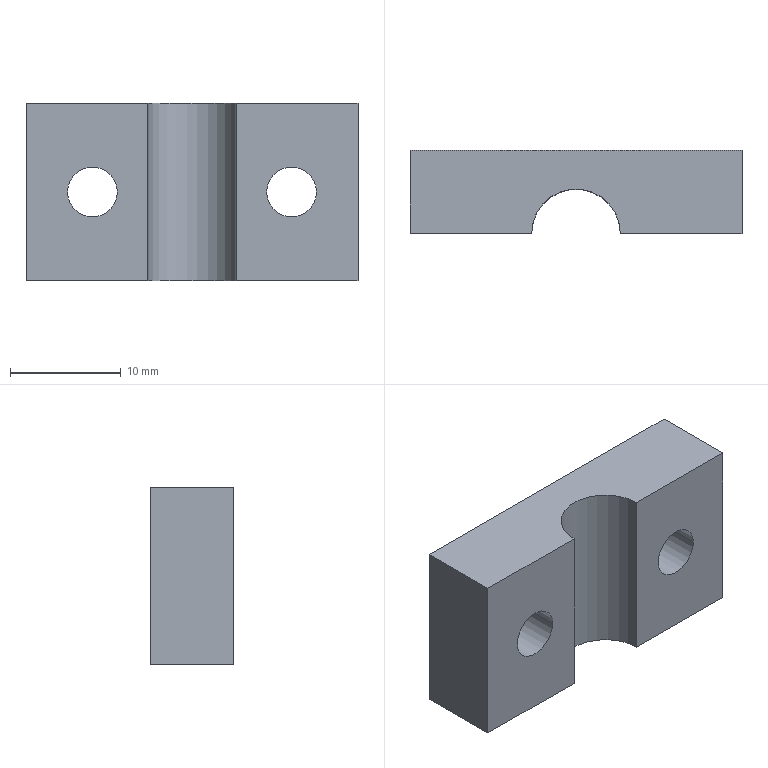Component | SolidWorks | JL001-05-03-1_JL001-05-01-012-1 | 1 solid | 12 faces | box 30 x 7.5 x 16 mm | volume 2959 mm3 | plane 7 | cylinder 5 | commonest cylinder face diameters 4.5 x4 8 x1
build123d program:
from build123d import *

# Parameters (mm, degrees)
SKETCH1_W                      = 16
SKETCH1_H                      = 30
BOSS_EXTRUDE1_DEPTH            = 7.5
SKETCH2_R                      = 4
CUT_EXTRUDE1_DEPTH             = 24.179
F_4_5_4_5_DIAMETER_HOLE1_D     = 4.5
F_4_5_4_5_DIAMETER_HOLE1_DEPTH = 10.1
F_4_5_4_5_DIAMETER_HOLE1_TIP   = 1.352


with BuildPart() as part:
    # Sketch1 → Boss-Extrude1 (new body)
    with BuildSketch(Plane(origin=(0, 0, 0), x_dir=(1, 0, 0), z_dir=(0, 1, 0))):
        Rectangle(SKETCH1_W, SKETCH1_H)
    extrude(amount=BOSS_EXTRUDE1_DEPTH)

    # Sketch2 → Cut-Extrude1 (cut, through all)
    with BuildSketch(Plane(origin=(8, 0, 0), x_dir=(0, 0, -1), z_dir=(1, 0, 0))):
        Circle(SKETCH2_R)
    extrude(amount=-CUT_EXTRUDE1_DEPTH, mode=Mode.SUBTRACT)

    # 4.5 _4.5_ Diameter Hole1
    with Locations(Plane(origin=(0, 7.5, 0), x_dir=(1, 0, 0), z_dir=(0, 1, 0))):
        with Locations((0, -9), (0, 9)):
            Hole(F_4_5_4_5_DIAMETER_HOLE1_D / 2, depth=F_4_5_4_5_DIAMETER_HOLE1_DEPTH)
            with Locations((0, 0, -(F_4_5_4_5_DIAMETER_HOLE1_DEPTH + F_4_5_4_5_DIAMETER_HOLE1_TIP / 2))):  # 118° drill point
                Cone(0, F_4_5_4_5_DIAMETER_HOLE1_D / 2, F_4_5_4_5_DIAMETER_HOLE1_TIP, mode=Mode.SUBTRACT)


solid = part.part

# Placed as in the assembly
solid = solid.moved(Location((0, 294.848, 85), (0, 90, 0)))
STEP:
#1=COLOUR_RGB('',0.7922,0.8196,0.9333);
#2=FILL_AREA_STYLE_COLOUR('',#1);
#3=FILL_AREA_STYLE('',(#2));
#4=SURFACE_STYLE_FILL_AREA(#3);
#5=SURFACE_SIDE_STYLE('',(#4));
#6=SURFACE_STYLE_USAGE(.BOTH.,#5);
#7=PRESENTATION_STYLE_ASSIGNMENT((#6));
#8=CARTESIAN_POINT('',(0.2657,11.608,3.346));
#9=VERTEX_POINT('',#8);
#10=CARTESIAN_POINT('',(0.4429,11.608,3.346));
#11=VERTEX_POINT('',#10);
#12=CARTESIAN_POINT('',(0.3543,11.608,3.346));
#13=DIRECTION('',(0.,1.,0.));
#14=DIRECTION('',(1.,0.,0.));
#15=AXIS2_PLACEMENT_3D('',#12,#13,#14);
#16=CIRCLE('',#15,0.08858);
#17=EDGE_CURVE('',#9,#11,#16,.T.);
#18=ORIENTED_EDGE('',*,*,#17,.F.);
#19=CARTESIAN_POINT('',(0.2657,11.903,3.346));
#20=VERTEX_POINT('',#19);
#21=CARTESIAN_POINT('',(0.2657,11.903,3.346));
#22=DIRECTION('',(0.,1.,0.));
#23=VECTOR('',#22,39.37);
#24=LINE('',#21,#23);
#25=EDGE_CURVE('',#9,#20,#24,.T.);
#26=ORIENTED_EDGE('',*,*,#25,.T.);
#27=CARTESIAN_POINT('',(0.4429,11.903,3.346));
#28=VERTEX_POINT('',#27);
#29=CARTESIAN_POINT('',(0.3543,11.903,3.346));
#30=DIRECTION('',(0.,1.,0.));
#31=DIRECTION('',(1.,0.,0.));
#32=AXIS2_PLACEMENT_3D('',#29,#30,#31);
#33=CIRCLE('',#32,0.08858);
#34=EDGE_CURVE('',#20,#28,#33,.T.);
#35=ORIENTED_EDGE('',*,*,#34,.T.);
#36=CARTESIAN_POINT('',(0.4429,11.903,3.346));
#37=DIRECTION('',(0.,1.,0.));
#38=VECTOR('',#37,39.37);
#39=LINE('',#36,#38);
#40=EDGE_CURVE('',#11,#28,#39,.T.);
#41=ORIENTED_EDGE('',*,*,#40,.F.);
#42=EDGE_LOOP('',(#18,#26,#35,#41));
#43=FACE_OUTER_BOUND('',#42,.T.);
#44=CARTESIAN_POINT('',(0.3543,11.903,3.346));
#45=DIRECTION('',(0.,1.,0.));
#46=DIRECTION('',(1.,0.,0.));
#47=AXIS2_PLACEMENT_3D('',#44,#45,#46);
#48=CYLINDRICAL_SURFACE('',#47,0.08858);
#49=ADVANCED_FACE('',(#43),#48,.F.);
#50=CARTESIAN_POINT('',(-0.4429,11.608,3.346));
#51=VERTEX_POINT('',#50);
#52=CARTESIAN_POINT('',(-0.2657,11.608,3.346));
#53=VERTEX_POINT('',#52);
#54=CARTESIAN_POINT('',(-0.3543,11.608,3.346));
#55=DIRECTION('',(0.,1.,0.));
#56=DIRECTION('',(1.,0.,0.));
#57=AXIS2_PLACEMENT_3D('',#54,#55,#56);
#58=CIRCLE('',#57,0.08858);
#59=EDGE_CURVE('',#51,#53,#58,.T.);
#60=ORIENTED_EDGE('',*,*,#59,.F.);
#61=CARTESIAN_POINT('',(-0.4429,11.903,3.346));
#62=VERTEX_POINT('',#61);
#63=CARTESIAN_POINT('',(-0.4429,11.903,3.346));
#64=DIRECTION('',(0.,1.,0.));
#65=VECTOR('',#64,39.37);
#66=LINE('',#63,#65);
#67=EDGE_CURVE('',#51,#62,#66,.T.);
#68=ORIENTED_EDGE('',*,*,#67,.T.);
#69=CARTESIAN_POINT('',(-0.2657,11.903,3.346));
#70=VERTEX_POINT('',#69);
#71=CARTESIAN_POINT('',(-0.3543,11.903,3.346));
#72=DIRECTION('',(0.,1.,0.));
#73=DIRECTION('',(1.,0.,0.));
#74=AXIS2_PLACEMENT_3D('',#71,#72,#73);
#75=CIRCLE('',#74,0.08858);
#76=EDGE_CURVE('',#62,#70,#75,.T.);
#77=ORIENTED_EDGE('',*,*,#76,.T.);
#78=CARTESIAN_POINT('',(-0.2657,11.903,3.346));
#79=DIRECTION('',(0.,1.,0.));
#80=VECTOR('',#79,39.37);
#81=LINE('',#78,#80);
#82=EDGE_CURVE('',#53,#70,#81,.T.);
#83=ORIENTED_EDGE('',*,*,#82,.F.);
#84=EDGE_LOOP('',(#60,#68,#77,#83));
#85=FACE_OUTER_BOUND('',#84,.T.);
#86=CARTESIAN_POINT('',(-0.3543,11.903,3.346));
#87=DIRECTION('',(0.,1.,0.));
#88=DIRECTION('',(1.,0.,0.));
#89=AXIS2_PLACEMENT_3D('',#86,#87,#88);
#90=CYLINDRICAL_SURFACE('',#89,0.08858);
#91=ADVANCED_FACE('',(#85),#90,.F.);
#92=CARTESIAN_POINT('',(0.3543,11.608,3.346));
#93=DIRECTION('',(0.,1.,0.));
#94=DIRECTION('',(1.,0.,0.));
#95=AXIS2_PLACEMENT_3D('',#92,#93,#94);
#96=CIRCLE('',#95,0.08858);
#97=EDGE_CURVE('',#11,#9,#96,.T.);
#98=ORIENTED_EDGE('',*,*,#97,.T.);
#99=ORIENTED_EDGE('',*,*,#17,.T.);
#100=EDGE_LOOP('',(#98,#99));
#101=FACE_BOUND('',#100,.T.);
#102=CARTESIAN_POINT('',(0.1575,11.608,3.661));
#103=VERTEX_POINT('',#102);
#104=CARTESIAN_POINT('',(0.5906,11.608,3.661));
#105=VERTEX_POINT('',#104);
#106=CARTESIAN_POINT('',(-0.5906,11.608,3.661));
#107=DIRECTION('',(1.,0.,-0.));
#108=VECTOR('',#107,39.37);
#109=LINE('',#106,#108);
#110=EDGE_CURVE('',#103,#105,#109,.T.);
#111=ORIENTED_EDGE('',*,*,#110,.F.);
#112=CARTESIAN_POINT('',(0.1575,11.608,3.031));
#113=VERTEX_POINT('',#112);
#114=CARTESIAN_POINT('',(0.1575,11.608,3.661));
#115=DIRECTION('',(-0.,0.,-1.));
#116=VECTOR('',#115,39.37);
#117=LINE('',#114,#116);
#118=EDGE_CURVE('',#103,#113,#117,.T.);
#119=ORIENTED_EDGE('',*,*,#118,.T.);
#120=CARTESIAN_POINT('',(0.5906,11.608,3.031));
#121=VERTEX_POINT('',#120);
#122=CARTESIAN_POINT('',(-0.5906,11.608,3.031));
#123=DIRECTION('',(-1.,0.,0.));
#124=VECTOR('',#123,39.37);
#125=LINE('',#122,#124);
#126=EDGE_CURVE('',#121,#113,#125,.T.);
#127=ORIENTED_EDGE('',*,*,#126,.F.);
#128=CARTESIAN_POINT('',(0.5906,11.608,3.661));
#129=DIRECTION('',(0.,0.,-1.));
#130=VECTOR('',#129,39.37);
#131=LINE('',#128,#130);
#132=EDGE_CURVE('',#105,#121,#131,.T.);
#133=ORIENTED_EDGE('',*,*,#132,.F.);
#134=EDGE_LOOP('',(#111,#119,#127,#133));
#135=FACE_OUTER_BOUND('',#134,.T.);
#136=CARTESIAN_POINT('',(-0.,11.608,3.346));
#137=DIRECTION('',(0.,1.,0.));
#138=DIRECTION('',(1.,0.,0.));
#139=AXIS2_PLACEMENT_3D('',#136,#137,#138);
#140=PLANE('',#139);
#141=ADVANCED_FACE('',(#101,#135),#140,.F.);
#142=ORIENTED_EDGE('',*,*,#126,.T.);
#143=CARTESIAN_POINT('',(-0.1575,11.608,3.031));
#144=VERTEX_POINT('',#143);
#145=CARTESIAN_POINT('',(-0.,11.608,3.031));
#146=DIRECTION('',(-0.,0.,-1.));
#147=DIRECTION('',(-1.,0.,0.));
#148=AXIS2_PLACEMENT_3D('',#145,#146,#147);
#149=CIRCLE('',#148,0.1575);
#150=EDGE_CURVE('',#144,#113,#149,.T.);
#151=ORIENTED_EDGE('',*,*,#150,.F.);
#152=CARTESIAN_POINT('',(-0.5906,11.608,3.031));
#153=VERTEX_POINT('',#152);
#154=CARTESIAN_POINT('',(-0.5906,11.608,3.031));
#155=DIRECTION('',(-1.,0.,0.));
#156=VECTOR('',#155,39.37);
#157=LINE('',#154,#156);
#158=EDGE_CURVE('',#144,#153,#157,.T.);
#159=ORIENTED_EDGE('',*,*,#158,.T.);
#160=CARTESIAN_POINT('',(-0.5906,11.903,3.031));
#161=VERTEX_POINT('',#160);
#162=CARTESIAN_POINT('',(-0.5906,11.903,3.031));
#163=DIRECTION('',(0.,-1.,0.));
#164=VECTOR('',#163,39.37);
#165=LINE('',#162,#164);
#166=EDGE_CURVE('',#161,#153,#165,.T.);
#167=ORIENTED_EDGE('',*,*,#166,.F.);
#168=CARTESIAN_POINT('',(0.5906,11.903,3.031));
#169=VERTEX_POINT('',#168);
#170=CARTESIAN_POINT('',(-0.5906,11.903,3.031));
#171=DIRECTION('',(-1.,0.,0.));
#172=VECTOR('',#171,39.37);
#173=LINE('',#170,#172);
#174=EDGE_CURVE('',#169,#161,#173,.T.);
#175=ORIENTED_EDGE('',*,*,#174,.F.);
#176=CARTESIAN_POINT('',(0.5906,11.903,3.031));
#177=DIRECTION('',(0.,-1.,0.));
#178=VECTOR('',#177,39.37);
#179=LINE('',#176,#178);
#180=EDGE_CURVE('',#169,#121,#179,.T.);
#181=ORIENTED_EDGE('',*,*,#180,.T.);
#182=EDGE_LOOP('',(#142,#151,#159,#167,#175,#181));
#183=FACE_OUTER_BOUND('',#182,.T.);
#184=CARTESIAN_POINT('',(-0.5906,11.903,3.031));
#185=DIRECTION('',(0.,0.,1.));
#186=DIRECTION('',(1.,0.,-0.));
#187=AXIS2_PLACEMENT_3D('',#184,#185,#186);
#188=PLANE('',#187);
#189=ADVANCED_FACE('',(#183),#188,.F.);
#190=CARTESIAN_POINT('',(-0.5906,11.608,3.661));
#191=VERTEX_POINT('',#190);
#192=CARTESIAN_POINT('',(-0.5906,11.608,3.661));
#193=DIRECTION('',(0.,0.,1.));
#194=VECTOR('',#193,39.37);
#195=LINE('',#192,#194);
#196=EDGE_CURVE('',#153,#191,#195,.T.);
#197=ORIENTED_EDGE('',*,*,#196,.T.);
#198=CARTESIAN_POINT('',(-0.5906,11.903,3.661));
#199=VERTEX_POINT('',#198);
#200=CARTESIAN_POINT('',(-0.5906,11.903,3.661));
#201=DIRECTION('',(0.,-1.,0.));
#202=VECTOR('',#201,39.37);
#203=LINE('',#200,#202);
#204=EDGE_CURVE('',#199,#191,#203,.T.);
#205=ORIENTED_EDGE('',*,*,#204,.F.);
#206=CARTESIAN_POINT('',(-0.5906,11.903,3.661));
#207=DIRECTION('',(0.,0.,1.));
#208=VECTOR('',#207,39.37);
#209=LINE('',#206,#208);
#210=EDGE_CURVE('',#161,#199,#209,.T.);
#211=ORIENTED_EDGE('',*,*,#210,.F.);
#212=ORIENTED_EDGE('',*,*,#166,.T.);
#213=EDGE_LOOP('',(#197,#205,#211,#212));
#214=FACE_OUTER_BOUND('',#213,.T.);
#215=CARTESIAN_POINT('',(-0.5906,11.903,3.661));
#216=DIRECTION('',(1.,0.,0.));
#217=DIRECTION('',(0.,0.,-1.));
#218=AXIS2_PLACEMENT_3D('',#215,#216,#217);
#219=PLANE('',#218);
#220=ADVANCED_FACE('',(#214),#219,.F.);
#221=CARTESIAN_POINT('',(-0.1575,11.608,3.661));
#222=VERTEX_POINT('',#221);
#223=CARTESIAN_POINT('',(-0.5906,11.608,3.661));
#224=DIRECTION('',(1.,0.,-0.));
#225=VECTOR('',#224,39.37);
#226=LINE('',#223,#225);
#227=EDGE_CURVE('',#191,#222,#226,.T.);
#228=ORIENTED_EDGE('',*,*,#227,.T.);
#229=CARTESIAN_POINT('',(-0.,11.608,3.661));
#230=DIRECTION('',(-0.,0.,-1.));
#231=DIRECTION('',(-1.,0.,0.));
#232=AXIS2_PLACEMENT_3D('',#229,#230,#231);
#233=CIRCLE('',#232,0.1575);
#234=EDGE_CURVE('',#222,#103,#233,.T.);
#235=ORIENTED_EDGE('',*,*,#234,.T.);
#236=ORIENTED_EDGE('',*,*,#110,.T.);
#237=CARTESIAN_POINT('',(0.5906,11.903,3.661));
#238=VERTEX_POINT('',#237);
#239=CARTESIAN_POINT('',(0.5906,11.903,3.661));
#240=DIRECTION('',(0.,-1.,0.));
#241=VECTOR('',#240,39.37);
#242=LINE('',#239,#241);
#243=EDGE_CURVE('',#238,#105,#242,.T.);
#244=ORIENTED_EDGE('',*,*,#243,.F.);
#245=CARTESIAN_POINT('',(-0.5906,11.903,3.661));
#246=DIRECTION('',(1.,0.,-0.));
#247=VECTOR('',#246,39.37);
#248=LINE('',#245,#247);
#249=EDGE_CURVE('',#199,#238,#248,.T.);
#250=ORIENTED_EDGE('',*,*,#249,.F.);
#251=ORIENTED_EDGE('',*,*,#204,.T.);
#252=EDGE_LOOP('',(#228,#235,#236,#244,#250,#251));
#253=FACE_OUTER_BOUND('',#252,.T.);
#254=CARTESIAN_POINT('',(-0.5906,11.903,3.661));
#255=DIRECTION('',(-0.,0.,-1.));
#256=DIRECTION('',(-1.,0.,0.));
#257=AXIS2_PLACEMENT_3D('',#254,#255,#256);
#258=PLANE('',#257);
#259=ADVANCED_FACE('',(#253),#258,.F.);
#260=ORIENTED_EDGE('',*,*,#132,.T.);
#261=ORIENTED_EDGE('',*,*,#180,.F.);
#262=CARTESIAN_POINT('',(0.5906,11.903,3.661));
#263=DIRECTION('',(0.,0.,-1.));
#264=VECTOR('',#263,39.37);
#265=LINE('',#262,#264);
#266=EDGE_CURVE('',#238,#169,#265,.T.);
#267=ORIENTED_EDGE('',*,*,#266,.F.);
#268=ORIENTED_EDGE('',*,*,#243,.T.);
#269=EDGE_LOOP('',(#260,#261,#267,#268));
#270=FACE_OUTER_BOUND('',#269,.T.);
#271=CARTESIAN_POINT('',(0.5906,11.903,3.661));
#272=DIRECTION('',(-1.,0.,0.));
#273=DIRECTION('',(0.,0.,1.));
#274=AXIS2_PLACEMENT_3D('',#271,#272,#273);
#275=PLANE('',#274);
#276=ADVANCED_FACE('',(#270),#275,.F.);
#277=CARTESIAN_POINT('',(0.3543,11.903,3.346));
#278=DIRECTION('',(0.,1.,0.));
#279=DIRECTION('',(1.,0.,0.));
#280=AXIS2_PLACEMENT_3D('',#277,#278,#279);
#281=CIRCLE('',#280,0.08858);
#282=EDGE_CURVE('',#28,#20,#281,.T.);
#283=ORIENTED_EDGE('',*,*,#282,.F.);
#284=ORIENTED_EDGE('',*,*,#34,.F.);
#285=EDGE_LOOP('',(#283,#284));
#286=FACE_BOUND('',#285,.T.);
#287=CARTESIAN_POINT('',(-0.3543,11.903,3.346));
#288=DIRECTION('',(0.,1.,0.));
#289=DIRECTION('',(1.,0.,0.));
#290=AXIS2_PLACEMENT_3D('',#287,#288,#289);
#291=CIRCLE('',#290,0.08858);
#292=EDGE_CURVE('',#70,#62,#291,.T.);
#293=ORIENTED_EDGE('',*,*,#292,.F.);
#294=ORIENTED_EDGE('',*,*,#76,.F.);
#295=EDGE_LOOP('',(#293,#294));
#296=FACE_BOUND('',#295,.T.);
#297=ORIENTED_EDGE('',*,*,#174,.T.);
#298=ORIENTED_EDGE('',*,*,#210,.T.);
#299=ORIENTED_EDGE('',*,*,#249,.T.);
#300=ORIENTED_EDGE('',*,*,#266,.T.);
#301=EDGE_LOOP('',(#297,#298,#299,#300));
#302=FACE_OUTER_BOUND('',#301,.T.);
#303=CARTESIAN_POINT('',(-0.,11.903,3.346));
#304=DIRECTION('',(0.,1.,0.));
#305=DIRECTION('',(1.,0.,0.));
#306=AXIS2_PLACEMENT_3D('',#303,#304,#305);
#307=PLANE('',#306);
#308=ADVANCED_FACE('',(#286,#296,#302),#307,.T.);
#309=CARTESIAN_POINT('',(-0.3543,11.608,3.346));
#310=DIRECTION('',(0.,1.,0.));
#311=DIRECTION('',(1.,0.,0.));
#312=AXIS2_PLACEMENT_3D('',#309,#310,#311);
#313=CIRCLE('',#312,0.08858);
#314=EDGE_CURVE('',#53,#51,#313,.T.);
#315=ORIENTED_EDGE('',*,*,#314,.T.);
#316=ORIENTED_EDGE('',*,*,#59,.T.);
#317=EDGE_LOOP('',(#315,#316));
#318=FACE_BOUND('',#317,.T.);
#319=ORIENTED_EDGE('',*,*,#158,.F.);
#320=CARTESIAN_POINT('',(-0.1575,11.608,3.661));
#321=DIRECTION('',(0.,0.,1.));
#322=VECTOR('',#321,39.37);
#323=LINE('',#320,#322);
#324=EDGE_CURVE('',#144,#222,#323,.T.);
#325=ORIENTED_EDGE('',*,*,#324,.T.);
#326=ORIENTED_EDGE('',*,*,#227,.F.);
#327=ORIENTED_EDGE('',*,*,#196,.F.);
#328=EDGE_LOOP('',(#319,#325,#326,#327));
#329=FACE_OUTER_BOUND('',#328,.T.);
#330=CARTESIAN_POINT('',(-0.,11.608,3.346));
#331=DIRECTION('',(0.,1.,0.));
#332=DIRECTION('',(1.,0.,0.));
#333=AXIS2_PLACEMENT_3D('',#330,#331,#332);
#334=PLANE('',#333);
#335=ADVANCED_FACE('',(#318,#329),#334,.F.);
#336=ORIENTED_EDGE('',*,*,#234,.F.);
#337=ORIENTED_EDGE('',*,*,#324,.F.);
#338=ORIENTED_EDGE('',*,*,#150,.T.);
#339=ORIENTED_EDGE('',*,*,#118,.F.);
#340=EDGE_LOOP('',(#336,#337,#338,#339));
#341=FACE_OUTER_BOUND('',#340,.T.);
#342=CARTESIAN_POINT('',(-0.,11.608,3.661));
#343=DIRECTION('',(-0.,0.,-1.));
#344=DIRECTION('',(-1.,0.,0.));
#345=AXIS2_PLACEMENT_3D('',#342,#343,#344);
#346=CYLINDRICAL_SURFACE('',#345,0.1575);
#347=ADVANCED_FACE('',(#341),#346,.F.);
#348=ORIENTED_EDGE('',*,*,#67,.F.);
#349=ORIENTED_EDGE('',*,*,#314,.F.);
#350=ORIENTED_EDGE('',*,*,#82,.T.);
#351=ORIENTED_EDGE('',*,*,#292,.T.);
#352=EDGE_LOOP('',(#348,#349,#350,#351));
#353=FACE_OUTER_BOUND('',#352,.T.);
#354=CARTESIAN_POINT('',(-0.3543,11.903,3.346));
#355=DIRECTION('',(0.,1.,0.));
#356=DIRECTION('',(1.,0.,0.));
#357=AXIS2_PLACEMENT_3D('',#354,#355,#356);
#358=CYLINDRICAL_SURFACE('',#357,0.08858);
#359=ADVANCED_FACE('',(#353),#358,.F.);
#360=ORIENTED_EDGE('',*,*,#25,.F.);
#361=ORIENTED_EDGE('',*,*,#97,.F.);
#362=ORIENTED_EDGE('',*,*,#40,.T.);
#363=ORIENTED_EDGE('',*,*,#282,.T.);
#364=EDGE_LOOP('',(#360,#361,#362,#363));
#365=FACE_OUTER_BOUND('',#364,.T.);
#366=CARTESIAN_POINT('',(0.3543,11.903,3.346));
#367=DIRECTION('',(0.,1.,0.));
#368=DIRECTION('',(1.,0.,0.));
#369=AXIS2_PLACEMENT_3D('',#366,#367,#368);
#370=CYLINDRICAL_SURFACE('',#369,0.08858);
#371=ADVANCED_FACE('',(#365),#370,.F.);
#372=CLOSED_SHELL('',(#49,#91,#141,#189,#220,#259,#276,#308,#335,#347,#359,#371));
#373=MANIFOLD_SOLID_BREP('',#372);
#374=STYLED_ITEM('',(#7),#373);
#375=PRESENTATION_LAYER_ASSIGNMENT('','',(#374));
#376=CARTESIAN_POINT('',(0.,0.,0.));
#377=DIRECTION('',(0.,0.,1.));
#378=DIRECTION('',(1.,0.,0.));
#379=AXIS2_PLACEMENT_3D('',#376,#377,#378);
#380=(LENGTH_UNIT()NAMED_UNIT(*)SI_UNIT($,.METRE.));
#381=LENGTH_MEASURE_WITH_UNIT(LENGTH_MEASURE(0.0254),#380);
#382=DIMENSIONAL_EXPONENTS(1.,0.,0.,0.,0.,0.,0.);
#383=(CONVERSION_BASED_UNIT('',#381)LENGTH_UNIT()NAMED_UNIT(#382));
#384=UNCERTAINTY_MEASURE_WITH_UNIT(LENGTH_MEASURE(0.00001),#383,'','');
#385=(NAMED_UNIT(*)PLANE_ANGLE_UNIT()SI_UNIT($,.RADIAN.));
#386=(NAMED_UNIT(*)SI_UNIT($,.STERADIAN.)SOLID_ANGLE_UNIT());
#387=(GEOMETRIC_REPRESENTATION_CONTEXT(3)GLOBAL_UNCERTAINTY_ASSIGNED_CONTEXT((#384))GLOBAL_UNIT_ASSIGNED_CONTEXT((#383,#385,#386))REPRESENTATION_CONTEXT('',''));
#388=ADVANCED_BREP_SHAPE_REPRESENTATION('',(#373,#379),#387);
#389=(LENGTH_UNIT()NAMED_UNIT(*)SI_UNIT($,.METRE.));
#390=LENGTH_MEASURE_WITH_UNIT(LENGTH_MEASURE(0.0254),#389);
#391=DIMENSIONAL_EXPONENTS(1.,0.,0.,0.,0.,0.,0.);
#392=(CONVERSION_BASED_UNIT('',#390)LENGTH_UNIT()NAMED_UNIT(#391));
#393=UNCERTAINTY_MEASURE_WITH_UNIT(LENGTH_MEASURE(0.00001),#392,'','');
#394=(NAMED_UNIT(*)PLANE_ANGLE_UNIT()SI_UNIT($,.RADIAN.));
#395=(NAMED_UNIT(*)SI_UNIT($,.STERADIAN.)SOLID_ANGLE_UNIT());
#396=(GEOMETRIC_REPRESENTATION_CONTEXT(3)GLOBAL_UNCERTAINTY_ASSIGNED_CONTEXT((#393))GLOBAL_UNIT_ASSIGNED_CONTEXT((#392,#394,#395))REPRESENTATION_CONTEXT('',''));
#397=MECHANICAL_DESIGN_GEOMETRIC_PRESENTATION_REPRESENTATION('',(#374),#396);